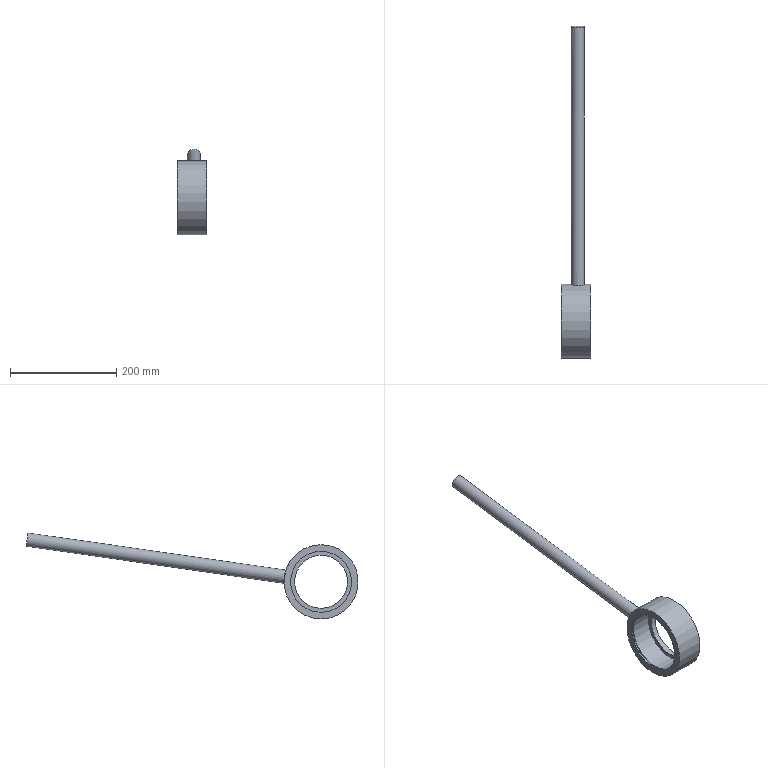Component | NX | DRIVE_ROD | 1 solid | 12 faces | box 55 x 626.09 x 161.96 mm | volume 538437 mm3 | cylinder 6 | plane 6 | commonest cylinder face diameters 115 x2 140 x1 100 x1 119 x1 25 x1
STEP:
#1=CARTESIAN_POINT('',(0.,0.,0.));
#2=DIRECTION('',(0.,0.,1.));
#3=DIRECTION('',(1.,0.,0.));
#4=AXIS2_PLACEMENT_3D('',#1,#2,#3);
#5=CARTESIAN_POINT('',(1368.754,222.349,548.477));
#6=VERTEX_POINT('',#5);
#7=CARTESIAN_POINT('',(1368.754,222.349,478.477));
#8=DIRECTION('',(1.,0.,0.));
#9=DIRECTION('',(0.,0.,1.));
#10=AXIS2_PLACEMENT_3D('',#7,#8,#9);
#11=CIRCLE('',#10,70.);
#12=CARTESIAN_POINT('',(1368.754,222.349,478.477));
#13=DIRECTION('',(-1.,0.,0.));
#14=DIRECTION('',(0.,0.,1.));
#15=AXIS2_PLACEMENT_3D('',#12,#13,#14);
#16=CYLINDRICAL_SURFACE('',#15,70.);
#17=CARTESIAN_POINT('',(6.283,0.));
#18=DIRECTION('',(-1.,0.));
#19=VECTOR('',#18,1.);
#20=LINE('',#17,#19);
#21=(GEOMETRIC_REPRESENTATION_CONTEXT(2)PARAMETRIC_REPRESENTATION_CONTEXT()REPRESENTATION_CONTEXT('',''));
#22=DEFINITIONAL_REPRESENTATION('',(#20),#21);
#23=PCURVE('',#16,#22);
#24=CARTESIAN_POINT('',(1368.754,222.349,478.477));
#25=DIRECTION('',(1.,0.,0.));
#26=DIRECTION('',(0.,0.,-1.));
#27=AXIS2_PLACEMENT_3D('',#24,#25,#26);
#28=PLANE('',#27);
#29=CARTESIAN_POINT('',(0.,0.));
#30=DIRECTION('',(-1.,0.));
#31=AXIS2_PLACEMENT_2D('',#29,#30);
#32=CIRCLE('',#31,70.);
#33=(GEOMETRIC_REPRESENTATION_CONTEXT(2)PARAMETRIC_REPRESENTATION_CONTEXT()REPRESENTATION_CONTEXT('',''));
#34=DEFINITIONAL_REPRESENTATION('',(#32),#33);
#35=PCURVE('',#28,#34);
#36=SURFACE_CURVE('',#11,(#23,#35),.PCURVE_S1.);
#37=EDGE_CURVE('',#6,#6,#36,.T.);
#38=ORIENTED_EDGE('',*,*,#37,.F.);
#39=CARTESIAN_POINT('',(1313.754,222.349,548.477));
#40=VERTEX_POINT('',#39);
#41=CARTESIAN_POINT('',(1368.754,222.349,548.477));
#42=CARTESIAN_POINT('',(1313.754,222.349,548.477));
#43=B_SPLINE_CURVE_WITH_KNOTS('',1,(#41,#42),.UNSPECIFIED.,.F.,.F.,(2,2),(0.,55.),.PIECEWISE_BEZIER_KNOTS.);
#44=CARTESIAN_POINT('',(6.283,0.));
#45=DIRECTION('',(0.,1.));
#46=VECTOR('',#45,1.);
#47=LINE('',#44,#46);
#48=(GEOMETRIC_REPRESENTATION_CONTEXT(2)PARAMETRIC_REPRESENTATION_CONTEXT()REPRESENTATION_CONTEXT('',''));
#49=DEFINITIONAL_REPRESENTATION('',(#47),#48);
#50=PCURVE('',#16,#49);
#51=CARTESIAN_POINT('',(0.,0.));
#52=DIRECTION('',(0.,1.));
#53=VECTOR('',#52,1.);
#54=LINE('',#51,#53);
#55=(GEOMETRIC_REPRESENTATION_CONTEXT(2)PARAMETRIC_REPRESENTATION_CONTEXT()REPRESENTATION_CONTEXT('',''));
#56=DEFINITIONAL_REPRESENTATION('',(#54),#55);
#57=PCURVE('',#16,#56);
#58=SEAM_CURVE('',#43,(#50,#57),.PCURVE_S1.);
#59=EDGE_CURVE('',#6,#40,#58,.T.);
#60=ORIENTED_EDGE('',*,*,#59,.T.);
#61=CARTESIAN_POINT('',(1313.754,222.349,478.477));
#62=DIRECTION('',(1.,0.,0.));
#63=DIRECTION('',(0.,0.,1.));
#64=AXIS2_PLACEMENT_3D('',#61,#62,#63);
#65=CIRCLE('',#64,70.);
#66=CARTESIAN_POINT('',(6.283,55.));
#67=DIRECTION('',(-1.,0.));
#68=VECTOR('',#67,1.);
#69=LINE('',#66,#68);
#70=(GEOMETRIC_REPRESENTATION_CONTEXT(2)PARAMETRIC_REPRESENTATION_CONTEXT()REPRESENTATION_CONTEXT('',''));
#71=DEFINITIONAL_REPRESENTATION('',(#69),#70);
#72=PCURVE('',#16,#71);
#73=CARTESIAN_POINT('',(1313.754,222.349,478.477));
#74=DIRECTION('',(1.,0.,0.));
#75=DIRECTION('',(0.,0.,-1.));
#76=AXIS2_PLACEMENT_3D('',#73,#74,#75);
#77=PLANE('',#76);
#78=CARTESIAN_POINT('',(0.,0.));
#79=DIRECTION('',(-1.,0.));
#80=AXIS2_PLACEMENT_2D('',#78,#79);
#81=CIRCLE('',#80,70.);
#82=(GEOMETRIC_REPRESENTATION_CONTEXT(2)PARAMETRIC_REPRESENTATION_CONTEXT()REPRESENTATION_CONTEXT('',''));
#83=DEFINITIONAL_REPRESENTATION('',(#81),#82);
#84=PCURVE('',#77,#83);
#85=SURFACE_CURVE('',#65,(#72,#84),.PCURVE_S1.);
#86=EDGE_CURVE('',#40,#40,#85,.T.);
#87=ORIENTED_EDGE('',*,*,#86,.T.);
#88=ORIENTED_EDGE('',*,*,#59,.F.);
#89=EDGE_LOOP('',(#38,#60,#87,#88));
#90=FACE_BOUND('',#89,.T.);
#91=CARTESIAN_POINT('',(1344.754,288.749,500.638));
#92=VERTEX_POINT('',#91);
#93=CARTESIAN_POINT('',(1341.444,288.749,500.638));
#94=CARTESIAN_POINT('',(1348.065,288.749,500.638));
#95=CARTESIAN_POINT('',(1351.293,289.212,499.33));
#96=CARTESIAN_POINT('',(1355.895,290.446,494.857));
#97=CARTESIAN_POINT('',(1357.252,291.173,491.667));
#98=CARTESIAN_POINT('',(1357.256,292.103,485.197));
#99=CARTESIAN_POINT('',(1355.921,292.303,481.944));
#100=CARTESIAN_POINT('',(1351.269,292.378,477.253));
#101=CARTESIAN_POINT('',(1348.026,292.302,475.893));
#102=CARTESIAN_POINT('',(1341.493,292.302,475.89));
#103=CARTESIAN_POINT('',(1338.23,292.378,477.267));
#104=CARTESIAN_POINT('',(1333.617,292.304,481.908));
#105=CARTESIAN_POINT('',(1332.257,292.109,485.146));
#106=CARTESIAN_POINT('',(1332.252,291.171,491.685));
#107=CARTESIAN_POINT('',(1333.611,290.447,494.851));
#108=CARTESIAN_POINT('',(1338.207,289.213,499.324));
#109=CARTESIAN_POINT('',(1341.444,288.749,500.638));
#110=CARTESIAN_POINT('',(1348.065,288.749,500.638));
#111=B_SPLINE_CURVE_WITH_KNOTS('',3,(#93,#94,#95,#96,#97,#98,#99,#100,#101,#102,#103,#104,#105,#106,#107,#108,#109,#110),.UNSPECIFIED.,.T.,.F.,(2,2,2,2,2,2,2,2,2,2,2),(-0.125,0.,0.125,0.25,0.375,0.5,0.625,0.75,0.875,1.,1.125),.UNSPECIFIED.);
#112=CARTESIAN_POINT('',(1.249,24.));
#113=CARTESIAN_POINT('',(1.249,23.398));
#114=CARTESIAN_POINT('',(1.25,22.2));
#115=CARTESIAN_POINT('',(1.256,20.449));
#116=CARTESIAN_POINT('',(1.265,18.775));
#117=CARTESIAN_POINT('',(1.277,17.21));
#118=CARTESIAN_POINT('',(1.292,15.782));
#119=CARTESIAN_POINT('',(1.311,14.524));
#120=CARTESIAN_POINT('',(1.331,13.462));
#121=CARTESIAN_POINT('',(1.354,12.609));
#122=CARTESIAN_POINT('',(1.378,11.98));
#123=CARTESIAN_POINT('',(1.403,11.591));
#124=CARTESIAN_POINT('',(1.428,11.455));
#125=CARTESIAN_POINT('',(1.454,11.587));
#126=CARTESIAN_POINT('',(1.478,11.972));
#127=CARTESIAN_POINT('',(1.502,12.596));
#128=CARTESIAN_POINT('',(1.525,13.448));
#129=CARTESIAN_POINT('',(1.546,14.515));
#130=CARTESIAN_POINT('',(1.564,15.788));
#131=CARTESIAN_POINT('',(1.579,17.226));
#132=CARTESIAN_POINT('',(1.592,18.799));
#133=CARTESIAN_POINT('',(1.601,20.472));
#134=CARTESIAN_POINT('',(1.606,22.215));
#135=CARTESIAN_POINT('',(1.608,23.995));
#136=CARTESIAN_POINT('',(1.606,25.777));
#137=CARTESIAN_POINT('',(1.601,27.523));
#138=CARTESIAN_POINT('',(1.592,29.199));
#139=CARTESIAN_POINT('',(1.579,30.772));
#140=CARTESIAN_POINT('',(1.564,32.208));
#141=CARTESIAN_POINT('',(1.546,33.469));
#142=CARTESIAN_POINT('',(1.525,34.533));
#143=CARTESIAN_POINT('',(1.503,35.388));
#144=CARTESIAN_POINT('',(1.479,36.018));
#145=CARTESIAN_POINT('',(1.454,36.409));
#146=CARTESIAN_POINT('',(1.428,36.545));
#147=CARTESIAN_POINT('',(1.403,36.411));
#148=CARTESIAN_POINT('',(1.378,36.023));
#149=CARTESIAN_POINT('',(1.354,35.395));
#150=CARTESIAN_POINT('',(1.331,34.542));
#151=CARTESIAN_POINT('',(1.311,33.481));
#152=CARTESIAN_POINT('',(1.293,32.225));
#153=CARTESIAN_POINT('',(1.277,30.796));
#154=CARTESIAN_POINT('',(1.265,29.229));
#155=CARTESIAN_POINT('',(1.256,27.553));
#156=CARTESIAN_POINT('',(1.25,25.801));
#157=CARTESIAN_POINT('',(1.249,24.602));
#158=CARTESIAN_POINT('',(1.249,24.));
#159=B_SPLINE_CURVE_WITH_KNOTS('',3,(#112,#113,#114,#115,#116,#117,#118,#119,#120,#121,#122,#123,#124,#125,#126,#127,#128,#129,#130,#131,#132,#133,#134,#135,#136,#137,#138,#139,#140,#141,#142,#143,#144,#145,#146,#147,#148,#149,#150,#151,#152,#153,#154,#155,#156,#157,#158),.UNSPECIFIED.,.T.,.F.,(4,1,1,1,1,1,1,1,1,1,1,1,1,1,1,1,1,1,1,1,1,1,1,1,1,1,1,1,1,1,1,1,1,1,1,1,1,1,1,1,1,1,1,1,4),(0.,0.02273,0.04545,0.06818,0.09091,0.1136,0.1364,0.1591,0.1818,0.2045,0.2273,0.25,0.2727,0.2955,0.3182,0.3409,0.3636,0.3864,0.4091,0.4318,0.4545,0.4773,0.5,0.5227,0.5455,0.5682,0.5909,0.6136,0.6364,0.6591,0.6818,0.7045,0.7273,0.75,0.7727,0.7955,0.8182,0.8409,0.8636,0.8864,0.9091,0.9318,0.9545,0.9773,1.),.QUASI_UNIFORM_KNOTS.);
#160=(GEOMETRIC_REPRESENTATION_CONTEXT(2)PARAMETRIC_REPRESENTATION_CONTEXT()REPRESENTATION_CONTEXT('',''));
#161=DEFINITIONAL_REPRESENTATION('',(#159),#160);
#162=PCURVE('',#16,#161);
#163=CARTESIAN_POINT('',(1344.754,776.666,558.06));
#164=DIRECTION('',(0.,0.9899,0.1421));
#165=DIRECTION('',(0.,-0.1421,0.9899));
#166=AXIS2_PLACEMENT_3D('',#163,#164,#165);
#167=CYLINDRICAL_SURFACE('',#166,12.5);
#168=CARTESIAN_POINT('',(0.,-491.125));
#169=CARTESIAN_POINT('',(0.04812,-491.125));
#170=CARTESIAN_POINT('',(0.144,-491.107));
#171=CARTESIAN_POINT('',(0.2872,-491.035));
#172=CARTESIAN_POINT('',(0.43,-490.928));
#173=CARTESIAN_POINT('',(0.5725,-490.793));
#174=CARTESIAN_POINT('',(0.7145,-490.641));
#175=CARTESIAN_POINT('',(0.8565,-490.479));
#176=CARTESIAN_POINT('',(0.9989,-490.328));
#177=CARTESIAN_POINT('',(1.142,-490.195));
#178=CARTESIAN_POINT('',(1.285,-490.089));
#179=CARTESIAN_POINT('',(1.428,-490.018));
#180=CARTESIAN_POINT('',(1.57,-489.991));
#181=CARTESIAN_POINT('',(1.713,-490.017));
#182=CARTESIAN_POINT('',(1.855,-490.087));
#183=CARTESIAN_POINT('',(1.998,-490.193));
#184=CARTESIAN_POINT('',(2.141,-490.326));
#185=CARTESIAN_POINT('',(2.284,-490.478));
#186=CARTESIAN_POINT('',(2.428,-490.642));
#187=CARTESIAN_POINT('',(2.571,-490.794));
#188=CARTESIAN_POINT('',(2.714,-490.929));
#189=CARTESIAN_POINT('',(2.856,-491.036));
#190=CARTESIAN_POINT('',(2.999,-491.107));
#191=CARTESIAN_POINT('',(3.141,-491.134));
#192=CARTESIAN_POINT('',(3.284,-491.107));
#193=CARTESIAN_POINT('',(3.427,-491.036));
#194=CARTESIAN_POINT('',(3.57,-490.928));
#195=CARTESIAN_POINT('',(3.713,-490.794));
#196=CARTESIAN_POINT('',(3.855,-490.642));
#197=CARTESIAN_POINT('',(3.997,-490.48));
#198=CARTESIAN_POINT('',(4.139,-490.329));
#199=CARTESIAN_POINT('',(4.282,-490.195));
#200=CARTESIAN_POINT('',(4.425,-490.089));
#201=CARTESIAN_POINT('',(4.568,-490.018));
#202=CARTESIAN_POINT('',(4.712,-489.991));
#203=CARTESIAN_POINT('',(4.855,-490.017));
#204=CARTESIAN_POINT('',(4.999,-490.088));
#205=CARTESIAN_POINT('',(5.141,-490.194));
#206=CARTESIAN_POINT('',(5.284,-490.328));
#207=CARTESIAN_POINT('',(5.426,-490.479));
#208=CARTESIAN_POINT('',(5.568,-490.64));
#209=CARTESIAN_POINT('',(5.71,-490.792));
#210=CARTESIAN_POINT('',(5.853,-490.927));
#211=CARTESIAN_POINT('',(5.996,-491.035));
#212=CARTESIAN_POINT('',(6.139,-491.107));
#213=CARTESIAN_POINT('',(6.235,-491.125));
#214=CARTESIAN_POINT('',(6.283,-491.125));
#215=B_SPLINE_CURVE_WITH_KNOTS('',3,(#168,#169,#170,#171,#172,#173,#174,#175,#176,#177,#178,#179,#180,#181,#182,#183,#184,#185,#186,#187,#188,#189,#190,#191,#192,#193,#194,#195,#196,#197,#198,#199,#200,#201,#202,#203,#204,#205,#206,#207,#208,#209,#210,#211,#212,#213,#214),.UNSPECIFIED.,.F.,.F.,(4,1,1,1,1,1,1,1,1,1,1,1,1,1,1,1,1,1,1,1,1,1,1,1,1,1,1,1,1,1,1,1,1,1,1,1,1,1,1,1,1,1,1,1,4),(0.,0.02273,0.04545,0.06818,0.09091,0.1136,0.1364,0.1591,0.1818,0.2045,0.2273,0.25,0.2727,0.2955,0.3182,0.3409,0.3636,0.3864,0.4091,0.4318,0.4545,0.4773,0.5,0.5227,0.5455,0.5682,0.5909,0.6136,0.6364,0.6591,0.6818,0.7045,0.7273,0.75,0.7727,0.7955,0.8182,0.8409,0.8636,0.8864,0.9091,0.9318,0.9545,0.9773,1.),.QUASI_UNIFORM_KNOTS.);
#216=(GEOMETRIC_REPRESENTATION_CONTEXT(2)PARAMETRIC_REPRESENTATION_CONTEXT()REPRESENTATION_CONTEXT('',''));
#217=DEFINITIONAL_REPRESENTATION('',(#215),#216);
#218=PCURVE('',#167,#217);
#219=SURFACE_CURVE('',#111,(#162,#218),.PCURVE_S1.);
#220=EDGE_CURVE('',#92,#92,#219,.T.);
#221=ORIENTED_EDGE('',*,*,#220,.F.);
#222=EDGE_LOOP('',(#221));
#223=FACE_BOUND('',#222,.T.);
#224=ADVANCED_FACE('',(#90,#223),#16,.T.);
#225=CARTESIAN_POINT('',(1358.754,222.349,420.977));
#226=VERTEX_POINT('',#225);
#227=CARTESIAN_POINT('',(1358.754,222.349,478.477));
#228=DIRECTION('',(1.,0.,0.));
#229=DIRECTION('',(0.,0.,-1.));
#230=AXIS2_PLACEMENT_3D('',#227,#228,#229);
#231=CIRCLE('',#230,57.5);
#232=CARTESIAN_POINT('',(1313.754,222.349,478.477));
#233=DIRECTION('',(1.,0.,0.));
#234=DIRECTION('',(0.,0.,-1.));
#235=AXIS2_PLACEMENT_3D('',#232,#233,#234);
#236=CYLINDRICAL_SURFACE('',#235,57.5);
#237=CARTESIAN_POINT('',(0.,45.));
#238=DIRECTION('',(1.,0.));
#239=VECTOR('',#238,1.);
#240=LINE('',#237,#239);
#241=(GEOMETRIC_REPRESENTATION_CONTEXT(2)PARAMETRIC_REPRESENTATION_CONTEXT()REPRESENTATION_CONTEXT('',''));
#242=DEFINITIONAL_REPRESENTATION('',(#240),#241);
#243=PCURVE('',#236,#242);
#244=CARTESIAN_POINT('',(1358.754,222.349,478.477));
#245=DIRECTION('',(1.,0.,0.));
#246=DIRECTION('',(0.,0.,-1.));
#247=AXIS2_PLACEMENT_3D('',#244,#245,#246);
#248=PLANE('',#247);
#249=CARTESIAN_POINT('',(0.,0.));
#250=DIRECTION('',(1.,0.));
#251=AXIS2_PLACEMENT_2D('',#249,#250);
#252=CIRCLE('',#251,57.5);
#253=(GEOMETRIC_REPRESENTATION_CONTEXT(2)PARAMETRIC_REPRESENTATION_CONTEXT()REPRESENTATION_CONTEXT('',''));
#254=DEFINITIONAL_REPRESENTATION('',(#252),#253);
#255=PCURVE('',#248,#254);
#256=SURFACE_CURVE('',#231,(#243,#255),.PCURVE_S1.);
#257=EDGE_CURVE('',#226,#226,#256,.T.);
#258=ORIENTED_EDGE('',*,*,#257,.F.);
#259=CARTESIAN_POINT('',(1318.754,222.349,420.977));
#260=VERTEX_POINT('',#259);
#261=CARTESIAN_POINT('',(1318.754,222.349,420.977));
#262=CARTESIAN_POINT('',(1358.754,222.349,420.977));
#263=B_SPLINE_CURVE_WITH_KNOTS('',1,(#261,#262),.UNSPECIFIED.,.F.,.F.,(2,2),(5.,45.),.PIECEWISE_BEZIER_KNOTS.);
#264=CARTESIAN_POINT('',(0.,0.));
#265=DIRECTION('',(0.,1.));
#266=VECTOR('',#265,1.);
#267=LINE('',#264,#266);
#268=(GEOMETRIC_REPRESENTATION_CONTEXT(2)PARAMETRIC_REPRESENTATION_CONTEXT()REPRESENTATION_CONTEXT('',''));
#269=DEFINITIONAL_REPRESENTATION('',(#267),#268);
#270=PCURVE('',#236,#269);
#271=CARTESIAN_POINT('',(6.283,0.));
#272=DIRECTION('',(0.,1.));
#273=VECTOR('',#272,1.);
#274=LINE('',#271,#273);
#275=(GEOMETRIC_REPRESENTATION_CONTEXT(2)PARAMETRIC_REPRESENTATION_CONTEXT()REPRESENTATION_CONTEXT('',''));
#276=DEFINITIONAL_REPRESENTATION('',(#274),#275);
#277=PCURVE('',#236,#276);
#278=SEAM_CURVE('',#263,(#270,#277),.PCURVE_S1.);
#279=EDGE_CURVE('',#260,#226,#278,.T.);
#280=ORIENTED_EDGE('',*,*,#279,.F.);
#281=CARTESIAN_POINT('',(1318.754,222.349,535.977));
#282=VERTEX_POINT('',#281);
#283=CARTESIAN_POINT('',(1318.754,222.349,478.477));
#284=DIRECTION('',(1.,0.,0.));
#285=DIRECTION('',(0.,0.,1.));
#286=AXIS2_PLACEMENT_3D('',#283,#284,#285);
#287=CIRCLE('',#286,57.5);
#288=CARTESIAN_POINT('',(-3.142,5.));
#289=DIRECTION('',(1.,0.));
#290=VECTOR('',#289,1.);
#291=LINE('',#288,#290);
#292=(GEOMETRIC_REPRESENTATION_CONTEXT(2)PARAMETRIC_REPRESENTATION_CONTEXT()REPRESENTATION_CONTEXT('',''));
#293=DEFINITIONAL_REPRESENTATION('',(#291),#292);
#294=PCURVE('',#236,#293);
#295=CARTESIAN_POINT('',(1318.754,222.349,478.477));
#296=DIRECTION('',(-1.,0.,0.));
#297=DIRECTION('',(0.,0.,1.));
#298=AXIS2_PLACEMENT_3D('',#295,#296,#297);
#299=PLANE('',#298);
#300=CARTESIAN_POINT('',(57.5,0.));
#301=CARTESIAN_POINT('',(57.5,-99.593));
#302=CARTESIAN_POINT('',(-28.75,-49.796));
#303=CARTESIAN_POINT('',(-115.,-0.));
#304=CARTESIAN_POINT('',(-28.75,49.796));
#305=CARTESIAN_POINT('',(57.5,99.593));
#306=CARTESIAN_POINT('',(57.5,0.));
#307=(BOUNDED_CURVE()B_SPLINE_CURVE(2,(#300,#301,#302,#303,#304,#305,#306),.UNSPECIFIED.,.T.,.F.)B_SPLINE_CURVE_WITH_KNOTS((1,2,2,2,2,1),(-2.094,0.,2.094,4.189,6.283,8.378),.UNSPECIFIED.)CURVE()GEOMETRIC_REPRESENTATION_ITEM()RATIONAL_B_SPLINE_CURVE((1.,0.5,1.,0.5,1.,0.5,1.))REPRESENTATION_ITEM(''));
#308=(GEOMETRIC_REPRESENTATION_CONTEXT(2)PARAMETRIC_REPRESENTATION_CONTEXT()REPRESENTATION_CONTEXT('',''));
#309=DEFINITIONAL_REPRESENTATION('',(#307),#308);
#310=PCURVE('',#299,#309);
#311=SURFACE_CURVE('',#287,(#294,#310),.PCURVE_S1.);
#312=EDGE_CURVE('',#260,#282,#311,.T.);
#313=ORIENTED_EDGE('',*,*,#312,.T.);
#314=CARTESIAN_POINT('',(1318.754,222.349,478.477));
#315=DIRECTION('',(1.,0.,0.));
#316=DIRECTION('',(0.,0.,1.));
#317=AXIS2_PLACEMENT_3D('',#314,#315,#316);
#318=CIRCLE('',#317,57.5);
#319=CARTESIAN_POINT('',(3.142,5.));
#320=DIRECTION('',(1.,0.));
#321=VECTOR('',#320,1.);
#322=LINE('',#319,#321);
#323=(GEOMETRIC_REPRESENTATION_CONTEXT(2)PARAMETRIC_REPRESENTATION_CONTEXT()REPRESENTATION_CONTEXT('',''));
#324=DEFINITIONAL_REPRESENTATION('',(#322),#323);
#325=PCURVE('',#236,#324);
#326=CARTESIAN_POINT('',(57.5,0.));
#327=CARTESIAN_POINT('',(57.5,-99.593));
#328=CARTESIAN_POINT('',(-28.75,-49.796));
#329=CARTESIAN_POINT('',(-115.,-0.));
#330=CARTESIAN_POINT('',(-28.75,49.796));
#331=CARTESIAN_POINT('',(57.5,99.593));
#332=CARTESIAN_POINT('',(57.5,0.));
#333=(BOUNDED_CURVE()B_SPLINE_CURVE(2,(#326,#327,#328,#329,#330,#331,#332),.UNSPECIFIED.,.T.,.F.)B_SPLINE_CURVE_WITH_KNOTS((1,2,2,2,2,1),(-2.094,0.,2.094,4.189,6.283,8.378),.UNSPECIFIED.)CURVE()GEOMETRIC_REPRESENTATION_ITEM()RATIONAL_B_SPLINE_CURVE((1.,0.5,1.,0.5,1.,0.5,1.))REPRESENTATION_ITEM(''));
#334=(GEOMETRIC_REPRESENTATION_CONTEXT(2)PARAMETRIC_REPRESENTATION_CONTEXT()REPRESENTATION_CONTEXT('',''));
#335=DEFINITIONAL_REPRESENTATION('',(#333),#334);
#336=PCURVE('',#299,#335);
#337=SURFACE_CURVE('',#318,(#325,#336),.PCURVE_S1.);
#338=EDGE_CURVE('',#282,#260,#337,.T.);
#339=ORIENTED_EDGE('',*,*,#338,.T.);
#340=ORIENTED_EDGE('',*,*,#279,.T.);
#341=EDGE_LOOP('',(#258,#280,#313,#339,#340));
#342=FACE_BOUND('',#341,.F.);
#343=ADVANCED_FACE('',(#342),#236,.F.);
#344=CARTESIAN_POINT('',(1358.754,222.349,428.477));
#345=VERTEX_POINT('',#344);
#346=CARTESIAN_POINT('',(1358.754,222.349,528.477));
#347=VERTEX_POINT('',#346);
#348=CARTESIAN_POINT('',(1358.754,222.349,478.477));
#349=DIRECTION('',(1.,0.,0.));
#350=DIRECTION('',(0.,0.,-1.));
#351=AXIS2_PLACEMENT_3D('',#348,#349,#350);
#352=CIRCLE('',#351,50.);
#353=CARTESIAN_POINT('',(1368.754,222.349,478.477));
#354=DIRECTION('',(-1.,0.,0.));
#355=DIRECTION('',(0.,0.,1.));
#356=AXIS2_PLACEMENT_3D('',#353,#354,#355);
#357=CYLINDRICAL_SURFACE('',#356,50.);
#358=CARTESIAN_POINT('',(3.142,10.));
#359=DIRECTION('',(-1.,0.));
#360=VECTOR('',#359,1.);
#361=LINE('',#358,#360);
#362=(GEOMETRIC_REPRESENTATION_CONTEXT(2)PARAMETRIC_REPRESENTATION_CONTEXT()REPRESENTATION_CONTEXT('',''));
#363=DEFINITIONAL_REPRESENTATION('',(#361),#362);
#364=PCURVE('',#357,#363);
#365=CARTESIAN_POINT('',(0.,0.));
#366=DIRECTION('',(1.,0.));
#367=AXIS2_PLACEMENT_2D('',#365,#366);
#368=CIRCLE('',#367,50.);
#369=(GEOMETRIC_REPRESENTATION_CONTEXT(2)PARAMETRIC_REPRESENTATION_CONTEXT()REPRESENTATION_CONTEXT('',''));
#370=DEFINITIONAL_REPRESENTATION('',(#368),#369);
#371=PCURVE('',#248,#370);
#372=SURFACE_CURVE('',#352,(#364,#371),.PCURVE_S1.);
#373=EDGE_CURVE('',#345,#347,#372,.T.);
#374=ORIENTED_EDGE('',*,*,#373,.T.);
#375=CARTESIAN_POINT('',(1368.754,222.349,528.477));
#376=VERTEX_POINT('',#375);
#377=CARTESIAN_POINT('',(1368.754,222.349,528.477));
#378=CARTESIAN_POINT('',(1358.754,222.349,528.477));
#379=B_SPLINE_CURVE_WITH_KNOTS('',1,(#377,#378),.UNSPECIFIED.,.F.,.F.,(2,2),(0.,10.),.PIECEWISE_BEZIER_KNOTS.);
#380=CARTESIAN_POINT('',(0.,0.));
#381=DIRECTION('',(0.,1.));
#382=VECTOR('',#381,1.);
#383=LINE('',#380,#382);
#384=(GEOMETRIC_REPRESENTATION_CONTEXT(2)PARAMETRIC_REPRESENTATION_CONTEXT()REPRESENTATION_CONTEXT('',''));
#385=DEFINITIONAL_REPRESENTATION('',(#383),#384);
#386=PCURVE('',#357,#385);
#387=CARTESIAN_POINT('',(6.283,0.));
#388=DIRECTION('',(0.,1.));
#389=VECTOR('',#388,1.);
#390=LINE('',#387,#389);
#391=(GEOMETRIC_REPRESENTATION_CONTEXT(2)PARAMETRIC_REPRESENTATION_CONTEXT()REPRESENTATION_CONTEXT('',''));
#392=DEFINITIONAL_REPRESENTATION('',(#390),#391);
#393=PCURVE('',#357,#392);
#394=SEAM_CURVE('',#379,(#386,#393),.PCURVE_S1.);
#395=EDGE_CURVE('',#376,#347,#394,.T.);
#396=ORIENTED_EDGE('',*,*,#395,.F.);
#397=CARTESIAN_POINT('',(1368.754,222.349,478.477));
#398=DIRECTION('',(1.,0.,0.));
#399=DIRECTION('',(0.,0.,1.));
#400=AXIS2_PLACEMENT_3D('',#397,#398,#399);
#401=CIRCLE('',#400,50.);
#402=CARTESIAN_POINT('',(6.283,0.));
#403=DIRECTION('',(-1.,0.));
#404=VECTOR('',#403,1.);
#405=LINE('',#402,#404);
#406=(GEOMETRIC_REPRESENTATION_CONTEXT(2)PARAMETRIC_REPRESENTATION_CONTEXT()REPRESENTATION_CONTEXT('',''));
#407=DEFINITIONAL_REPRESENTATION('',(#405),#406);
#408=PCURVE('',#357,#407);
#409=CARTESIAN_POINT('',(0.,0.));
#410=DIRECTION('',(-1.,0.));
#411=AXIS2_PLACEMENT_2D('',#409,#410);
#412=CIRCLE('',#411,50.);
#413=(GEOMETRIC_REPRESENTATION_CONTEXT(2)PARAMETRIC_REPRESENTATION_CONTEXT()REPRESENTATION_CONTEXT('',''));
#414=DEFINITIONAL_REPRESENTATION('',(#412),#413);
#415=PCURVE('',#28,#414);
#416=SURFACE_CURVE('',#401,(#408,#415),.PCURVE_S1.);
#417=EDGE_CURVE('',#376,#376,#416,.T.);
#418=ORIENTED_EDGE('',*,*,#417,.F.);
#419=ORIENTED_EDGE('',*,*,#395,.T.);
#420=CARTESIAN_POINT('',(1358.754,222.349,478.477));
#421=DIRECTION('',(1.,0.,0.));
#422=DIRECTION('',(0.,0.,-1.));
#423=AXIS2_PLACEMENT_3D('',#420,#421,#422);
#424=CIRCLE('',#423,50.);
#425=CARTESIAN_POINT('',(9.425,10.));
#426=DIRECTION('',(-1.,0.));
#427=VECTOR('',#426,1.);
#428=LINE('',#425,#427);
#429=(GEOMETRIC_REPRESENTATION_CONTEXT(2)PARAMETRIC_REPRESENTATION_CONTEXT()REPRESENTATION_CONTEXT('',''));
#430=DEFINITIONAL_REPRESENTATION('',(#428),#429);
#431=PCURVE('',#357,#430);
#432=CARTESIAN_POINT('',(0.,0.));
#433=DIRECTION('',(1.,0.));
#434=AXIS2_PLACEMENT_2D('',#432,#433);
#435=CIRCLE('',#434,50.);
#436=(GEOMETRIC_REPRESENTATION_CONTEXT(2)PARAMETRIC_REPRESENTATION_CONTEXT()REPRESENTATION_CONTEXT('',''));
#437=DEFINITIONAL_REPRESENTATION('',(#435),#436);
#438=PCURVE('',#248,#437);
#439=SURFACE_CURVE('',#424,(#431,#438),.PCURVE_S1.);
#440=EDGE_CURVE('',#347,#345,#439,.T.);
#441=ORIENTED_EDGE('',*,*,#440,.T.);
#442=EDGE_LOOP('',(#374,#396,#418,#419,#441));
#443=FACE_BOUND('',#442,.F.);
#444=ADVANCED_FACE('',(#443),#357,.F.);
#445=ORIENTED_EDGE('',*,*,#37,.T.);
#446=EDGE_LOOP('',(#445));
#447=FACE_BOUND('',#446,.T.);
#448=ORIENTED_EDGE('',*,*,#417,.F.);
#449=EDGE_LOOP('',(#448));
#450=FACE_BOUND('',#449,.T.);
#451=ADVANCED_FACE('',(#447,#450),#28,.T.);
#452=CARTESIAN_POINT('',(1313.754,222.349,420.977));
#453=VERTEX_POINT('',#452);
#454=CARTESIAN_POINT('',(1313.754,222.349,478.477));
#455=DIRECTION('',(1.,0.,0.));
#456=DIRECTION('',(0.,0.,-1.));
#457=AXIS2_PLACEMENT_3D('',#454,#455,#456);
#458=CIRCLE('',#457,57.5);
#459=CARTESIAN_POINT('',(0.,0.));
#460=DIRECTION('',(1.,0.));
#461=AXIS2_PLACEMENT_2D('',#459,#460);
#462=CIRCLE('',#461,57.5);
#463=(GEOMETRIC_REPRESENTATION_CONTEXT(2)PARAMETRIC_REPRESENTATION_CONTEXT()REPRESENTATION_CONTEXT('',''));
#464=DEFINITIONAL_REPRESENTATION('',(#462),#463);
#465=PCURVE('',#77,#464);
#466=CARTESIAN_POINT('',(1313.754,222.349,478.477));
#467=DIRECTION('',(1.,0.,0.));
#468=DIRECTION('',(0.,0.,-1.));
#469=AXIS2_PLACEMENT_3D('',#466,#467,#468);
#470=CYLINDRICAL_SURFACE('',#469,57.5);
#471=CARTESIAN_POINT('',(0.,0.));
#472=DIRECTION('',(1.,0.));
#473=VECTOR('',#472,1.);
#474=LINE('',#471,#473);
#475=(GEOMETRIC_REPRESENTATION_CONTEXT(2)PARAMETRIC_REPRESENTATION_CONTEXT()REPRESENTATION_CONTEXT('',''));
#476=DEFINITIONAL_REPRESENTATION('',(#474),#475);
#477=PCURVE('',#470,#476);
#478=SURFACE_CURVE('',#458,(#465,#477),.PCURVE_S1.);
#479=EDGE_CURVE('',#453,#453,#478,.T.);
#480=ORIENTED_EDGE('',*,*,#479,.T.);
#481=EDGE_LOOP('',(#480));
#482=FACE_BOUND('',#481,.T.);
#483=ORIENTED_EDGE('',*,*,#86,.F.);
#484=EDGE_LOOP('',(#483));
#485=FACE_BOUND('',#484,.T.);
#486=ADVANCED_FACE('',(#482,#485),#77,.F.);
#487=ORIENTED_EDGE('',*,*,#373,.T.);
#488=ORIENTED_EDGE('',*,*,#440,.T.);
#489=EDGE_LOOP('',(#487,#488));
#490=FACE_BOUND('',#489,.T.);
#491=ORIENTED_EDGE('',*,*,#257,.F.);
#492=EDGE_LOOP('',(#491));
#493=FACE_BOUND('',#492,.T.);
#494=ADVANCED_FACE('',(#490,#493),#248,.F.);
#495=CARTESIAN_POINT('',(1314.754,222.349,420.977));
#496=VERTEX_POINT('',#495);
#497=CARTESIAN_POINT('',(1314.754,222.349,535.977));
#498=VERTEX_POINT('',#497);
#499=CARTESIAN_POINT('',(1314.754,222.349,478.477));
#500=DIRECTION('',(1.,0.,0.));
#501=DIRECTION('',(0.,0.,1.));
#502=AXIS2_PLACEMENT_3D('',#499,#500,#501);
#503=CIRCLE('',#502,57.5);
#504=CARTESIAN_POINT('',(-3.142,1.));
#505=DIRECTION('',(1.,0.));
#506=VECTOR('',#505,1.);
#507=LINE('',#504,#506);
#508=(GEOMETRIC_REPRESENTATION_CONTEXT(2)PARAMETRIC_REPRESENTATION_CONTEXT()REPRESENTATION_CONTEXT('',''));
#509=DEFINITIONAL_REPRESENTATION('',(#507),#508);
#510=PCURVE('',#470,#509);
#511=CARTESIAN_POINT('',(1314.754,222.349,478.477));
#512=DIRECTION('',(-1.,0.,0.));
#513=DIRECTION('',(0.,0.,1.));
#514=AXIS2_PLACEMENT_3D('',#511,#512,#513);
#515=PLANE('',#514);
#516=CARTESIAN_POINT('',(57.5,0.));
#517=CARTESIAN_POINT('',(57.5,-99.593));
#518=CARTESIAN_POINT('',(-28.75,-49.796));
#519=CARTESIAN_POINT('',(-115.,-0.));
#520=CARTESIAN_POINT('',(-28.75,49.796));
#521=CARTESIAN_POINT('',(57.5,99.593));
#522=CARTESIAN_POINT('',(57.5,0.));
#523=(BOUNDED_CURVE()B_SPLINE_CURVE(2,(#516,#517,#518,#519,#520,#521,#522),.UNSPECIFIED.,.T.,.F.)B_SPLINE_CURVE_WITH_KNOTS((1,2,2,2,2,1),(-2.094,0.,2.094,4.189,6.283,8.378),.UNSPECIFIED.)CURVE()GEOMETRIC_REPRESENTATION_ITEM()RATIONAL_B_SPLINE_CURVE((1.,0.5,1.,0.5,1.,0.5,1.))REPRESENTATION_ITEM(''));
#524=(GEOMETRIC_REPRESENTATION_CONTEXT(2)PARAMETRIC_REPRESENTATION_CONTEXT()REPRESENTATION_CONTEXT('',''));
#525=DEFINITIONAL_REPRESENTATION('',(#523),#524);
#526=PCURVE('',#515,#525);
#527=SURFACE_CURVE('',#503,(#510,#526),.PCURVE_S1.);
#528=EDGE_CURVE('',#496,#498,#527,.T.);
#529=ORIENTED_EDGE('',*,*,#528,.F.);
#530=CARTESIAN_POINT('',(1313.754,222.349,420.977));
#531=CARTESIAN_POINT('',(1314.754,222.349,420.977));
#532=B_SPLINE_CURVE_WITH_KNOTS('',1,(#530,#531),.UNSPECIFIED.,.F.,.F.,(2,2),(0.,1.),.PIECEWISE_BEZIER_KNOTS.);
#533=CARTESIAN_POINT('',(0.,0.));
#534=DIRECTION('',(0.,1.));
#535=VECTOR('',#534,1.);
#536=LINE('',#533,#535);
#537=(GEOMETRIC_REPRESENTATION_CONTEXT(2)PARAMETRIC_REPRESENTATION_CONTEXT()REPRESENTATION_CONTEXT('',''));
#538=DEFINITIONAL_REPRESENTATION('',(#536),#537);
#539=PCURVE('',#470,#538);
#540=CARTESIAN_POINT('',(6.283,0.));
#541=DIRECTION('',(0.,1.));
#542=VECTOR('',#541,1.);
#543=LINE('',#540,#542);
#544=(GEOMETRIC_REPRESENTATION_CONTEXT(2)PARAMETRIC_REPRESENTATION_CONTEXT()REPRESENTATION_CONTEXT('',''));
#545=DEFINITIONAL_REPRESENTATION('',(#543),#544);
#546=PCURVE('',#470,#545);
#547=SEAM_CURVE('',#532,(#539,#546),.PCURVE_S1.);
#548=EDGE_CURVE('',#453,#496,#547,.T.);
#549=ORIENTED_EDGE('',*,*,#548,.F.);
#550=ORIENTED_EDGE('',*,*,#479,.T.);
#551=ORIENTED_EDGE('',*,*,#548,.T.);
#552=CARTESIAN_POINT('',(1314.754,222.349,478.477));
#553=DIRECTION('',(1.,0.,0.));
#554=DIRECTION('',(0.,0.,1.));
#555=AXIS2_PLACEMENT_3D('',#552,#553,#554);
#556=CIRCLE('',#555,57.5);
#557=CARTESIAN_POINT('',(3.142,1.));
#558=DIRECTION('',(1.,0.));
#559=VECTOR('',#558,1.);
#560=LINE('',#557,#559);
#561=(GEOMETRIC_REPRESENTATION_CONTEXT(2)PARAMETRIC_REPRESENTATION_CONTEXT()REPRESENTATION_CONTEXT('',''));
#562=DEFINITIONAL_REPRESENTATION('',(#560),#561);
#563=PCURVE('',#470,#562);
#564=CARTESIAN_POINT('',(57.5,0.));
#565=CARTESIAN_POINT('',(57.5,-99.593));
#566=CARTESIAN_POINT('',(-28.75,-49.796));
#567=CARTESIAN_POINT('',(-115.,-0.));
#568=CARTESIAN_POINT('',(-28.75,49.796));
#569=CARTESIAN_POINT('',(57.5,99.593));
#570=CARTESIAN_POINT('',(57.5,0.));
#571=(BOUNDED_CURVE()B_SPLINE_CURVE(2,(#564,#565,#566,#567,#568,#569,#570),.UNSPECIFIED.,.T.,.F.)B_SPLINE_CURVE_WITH_KNOTS((1,2,2,2,2,1),(-2.094,0.,2.094,4.189,6.283,8.378),.UNSPECIFIED.)CURVE()GEOMETRIC_REPRESENTATION_ITEM()RATIONAL_B_SPLINE_CURVE((1.,0.5,1.,0.5,1.,0.5,1.))REPRESENTATION_ITEM(''));
#572=(GEOMETRIC_REPRESENTATION_CONTEXT(2)PARAMETRIC_REPRESENTATION_CONTEXT()REPRESENTATION_CONTEXT('',''));
#573=DEFINITIONAL_REPRESENTATION('',(#571),#572);
#574=PCURVE('',#515,#573);
#575=SURFACE_CURVE('',#556,(#563,#574),.PCURVE_S1.);
#576=EDGE_CURVE('',#498,#496,#575,.T.);
#577=ORIENTED_EDGE('',*,*,#576,.F.);
#578=EDGE_LOOP('',(#529,#549,#550,#551,#577));
#579=FACE_BOUND('',#578,.F.);
#580=ADVANCED_FACE('',(#579),#470,.F.);
#581=CARTESIAN_POINT('',(1318.754,281.849,478.477));
#582=VERTEX_POINT('',#581);
#583=CARTESIAN_POINT('',(1318.754,222.349,478.477));
#584=DIRECTION('',(1.,0.,0.));
#585=DIRECTION('',(0.,1.,0.));
#586=AXIS2_PLACEMENT_3D('',#583,#584,#585);
#587=CIRCLE('',#586,59.5);
#588=CARTESIAN_POINT('',(0.,59.5));
#589=CARTESIAN_POINT('',(103.057,59.5));
#590=CARTESIAN_POINT('',(51.529,-29.75));
#591=CARTESIAN_POINT('',(0.,-119.));
#592=CARTESIAN_POINT('',(-51.529,-29.75));
#593=CARTESIAN_POINT('',(-103.057,59.5));
#594=CARTESIAN_POINT('',(0.,59.5));
#595=(BOUNDED_CURVE()B_SPLINE_CURVE(2,(#588,#589,#590,#591,#592,#593,#594),.UNSPECIFIED.,.T.,.F.)B_SPLINE_CURVE_WITH_KNOTS((1,2,2,2,2,1),(-2.094,0.,2.094,4.189,6.283,8.378),.UNSPECIFIED.)CURVE()GEOMETRIC_REPRESENTATION_ITEM()RATIONAL_B_SPLINE_CURVE((1.,0.5,1.,0.5,1.,0.5,1.))REPRESENTATION_ITEM(''));
#596=(GEOMETRIC_REPRESENTATION_CONTEXT(2)PARAMETRIC_REPRESENTATION_CONTEXT()REPRESENTATION_CONTEXT('',''));
#597=DEFINITIONAL_REPRESENTATION('',(#595),#596);
#598=PCURVE('',#299,#597);
#599=CARTESIAN_POINT('',(1318.754,222.349,478.477));
#600=DIRECTION('',(-1.,0.,0.));
#601=DIRECTION('',(0.,0.,1.));
#602=AXIS2_PLACEMENT_3D('',#599,#600,#601);
#603=CYLINDRICAL_SURFACE('',#602,59.5);
#604=CARTESIAN_POINT('',(7.854,0.));
#605=DIRECTION('',(-1.,0.));
#606=VECTOR('',#605,1.);
#607=LINE('',#604,#606);
#608=(GEOMETRIC_REPRESENTATION_CONTEXT(2)PARAMETRIC_REPRESENTATION_CONTEXT()REPRESENTATION_CONTEXT('',''));
#609=DEFINITIONAL_REPRESENTATION('',(#607),#608);
#610=PCURVE('',#603,#609);
#611=SURFACE_CURVE('',#587,(#598,#610),.PCURVE_S1.);
#612=EDGE_CURVE('',#582,#582,#611,.T.);
#613=ORIENTED_EDGE('',*,*,#612,.F.);
#614=EDGE_LOOP('',(#613));
#615=FACE_BOUND('',#614,.T.);
#616=ORIENTED_EDGE('',*,*,#338,.T.);
#617=ORIENTED_EDGE('',*,*,#312,.T.);
#618=EDGE_LOOP('',(#616,#617));
#619=FACE_BOUND('',#618,.T.);
#620=ADVANCED_FACE('',(#615,#619),#299,.T.);
#621=CARTESIAN_POINT('',(1314.754,281.849,478.477));
#622=VERTEX_POINT('',#621);
#623=CARTESIAN_POINT('',(1314.754,222.349,478.477));
#624=DIRECTION('',(1.,0.,0.));
#625=DIRECTION('',(0.,1.,0.));
#626=AXIS2_PLACEMENT_3D('',#623,#624,#625);
#627=CIRCLE('',#626,59.5);
#628=CARTESIAN_POINT('',(0.,59.5));
#629=CARTESIAN_POINT('',(103.057,59.5));
#630=CARTESIAN_POINT('',(51.529,-29.75));
#631=CARTESIAN_POINT('',(0.,-119.));
#632=CARTESIAN_POINT('',(-51.529,-29.75));
#633=CARTESIAN_POINT('',(-103.057,59.5));
#634=CARTESIAN_POINT('',(0.,59.5));
#635=(BOUNDED_CURVE()B_SPLINE_CURVE(2,(#628,#629,#630,#631,#632,#633,#634),.UNSPECIFIED.,.T.,.F.)B_SPLINE_CURVE_WITH_KNOTS((1,2,2,2,2,1),(-2.094,0.,2.094,4.189,6.283,8.378),.UNSPECIFIED.)CURVE()GEOMETRIC_REPRESENTATION_ITEM()RATIONAL_B_SPLINE_CURVE((1.,0.5,1.,0.5,1.,0.5,1.))REPRESENTATION_ITEM(''));
#636=(GEOMETRIC_REPRESENTATION_CONTEXT(2)PARAMETRIC_REPRESENTATION_CONTEXT()REPRESENTATION_CONTEXT('',''));
#637=DEFINITIONAL_REPRESENTATION('',(#635),#636);
#638=PCURVE('',#515,#637);
#639=CARTESIAN_POINT('',(7.854,4.));
#640=DIRECTION('',(-1.,0.));
#641=VECTOR('',#640,1.);
#642=LINE('',#639,#641);
#643=(GEOMETRIC_REPRESENTATION_CONTEXT(2)PARAMETRIC_REPRESENTATION_CONTEXT()REPRESENTATION_CONTEXT('',''));
#644=DEFINITIONAL_REPRESENTATION('',(#642),#643);
#645=PCURVE('',#603,#644);
#646=SURFACE_CURVE('',#627,(#638,#645),.PCURVE_S1.);
#647=EDGE_CURVE('',#622,#622,#646,.T.);
#648=ORIENTED_EDGE('',*,*,#647,.T.);
#649=EDGE_LOOP('',(#648));
#650=FACE_BOUND('',#649,.T.);
#651=ORIENTED_EDGE('',*,*,#576,.F.);
#652=ORIENTED_EDGE('',*,*,#528,.F.);
#653=EDGE_LOOP('',(#651,#652));
#654=FACE_BOUND('',#653,.T.);
#655=ADVANCED_FACE('',(#650,#654),#515,.F.);
#656=ORIENTED_EDGE('',*,*,#612,.F.);
#657=CARTESIAN_POINT('',(1318.754,281.849,478.477));
#658=CARTESIAN_POINT('',(1314.754,281.849,478.477));
#659=B_SPLINE_CURVE_WITH_KNOTS('',1,(#657,#658),.UNSPECIFIED.,.F.,.F.,(2,2),(0.,4.),.PIECEWISE_BEZIER_KNOTS.);
#660=CARTESIAN_POINT('',(7.854,0.));
#661=DIRECTION('',(0.,1.));
#662=VECTOR('',#661,1.);
#663=LINE('',#660,#662);
#664=(GEOMETRIC_REPRESENTATION_CONTEXT(2)PARAMETRIC_REPRESENTATION_CONTEXT()REPRESENTATION_CONTEXT('',''));
#665=DEFINITIONAL_REPRESENTATION('',(#663),#664);
#666=PCURVE('',#603,#665);
#667=CARTESIAN_POINT('',(1.571,0.));
#668=DIRECTION('',(0.,1.));
#669=VECTOR('',#668,1.);
#670=LINE('',#667,#669);
#671=(GEOMETRIC_REPRESENTATION_CONTEXT(2)PARAMETRIC_REPRESENTATION_CONTEXT()REPRESENTATION_CONTEXT('',''));
#672=DEFINITIONAL_REPRESENTATION('',(#670),#671);
#673=PCURVE('',#603,#672);
#674=SEAM_CURVE('',#659,(#666,#673),.PCURVE_S1.);
#675=EDGE_CURVE('',#582,#622,#674,.T.);
#676=ORIENTED_EDGE('',*,*,#675,.T.);
#677=ORIENTED_EDGE('',*,*,#647,.T.);
#678=ORIENTED_EDGE('',*,*,#675,.F.);
#679=EDGE_LOOP('',(#656,#676,#677,#678));
#680=FACE_BOUND('',#679,.F.);
#681=ADVANCED_FACE('',(#680),#603,.F.);
#682=CARTESIAN_POINT('',(1344.754,774.889,570.433));
#683=VERTEX_POINT('',#682);
#684=CARTESIAN_POINT('',(1344.754,776.666,558.06));
#685=DIRECTION('',(0.,0.9899,0.1421));
#686=DIRECTION('',(0.,-0.1421,0.9899));
#687=AXIS2_PLACEMENT_3D('',#684,#685,#686);
#688=CIRCLE('',#687,12.5);
#689=CARTESIAN_POINT('',(0.,-0.));
#690=DIRECTION('',(1.,0.));
#691=VECTOR('',#690,1.);
#692=LINE('',#689,#691);
#693=(GEOMETRIC_REPRESENTATION_CONTEXT(2)PARAMETRIC_REPRESENTATION_CONTEXT()REPRESENTATION_CONTEXT('',''));
#694=DEFINITIONAL_REPRESENTATION('',(#692),#693);
#695=PCURVE('',#167,#694);
#696=CARTESIAN_POINT('',(1344.754,776.666,558.06));
#697=DIRECTION('',(0.,0.9899,0.1421));
#698=DIRECTION('',(0.,-0.1421,0.9899));
#699=AXIS2_PLACEMENT_3D('',#696,#697,#698);
#700=PLANE('',#699);
#701=CARTESIAN_POINT('',(0.,0.));
#702=DIRECTION('',(1.,0.));
#703=AXIS2_PLACEMENT_2D('',#701,#702);
#704=CIRCLE('',#703,12.5);
#705=(GEOMETRIC_REPRESENTATION_CONTEXT(2)PARAMETRIC_REPRESENTATION_CONTEXT()REPRESENTATION_CONTEXT('',''));
#706=DEFINITIONAL_REPRESENTATION('',(#704),#705);
#707=PCURVE('',#700,#706);
#708=SURFACE_CURVE('',#688,(#695,#707),.PCURVE_S1.);
#709=EDGE_CURVE('',#683,#683,#708,.T.);
#710=ORIENTED_EDGE('',*,*,#709,.F.);
#711=CARTESIAN_POINT('',(1344.754,288.749,500.638));
#712=CARTESIAN_POINT('',(1344.754,774.889,570.433));
#713=B_SPLINE_CURVE_WITH_KNOTS('',1,(#711,#712),.UNSPECIFIED.,.F.,.F.,(2,2),(-491.125,-0.),.PIECEWISE_BEZIER_KNOTS.);
#714=CARTESIAN_POINT('',(0.,0.));
#715=DIRECTION('',(0.,1.));
#716=VECTOR('',#715,1.);
#717=LINE('',#714,#716);
#718=(GEOMETRIC_REPRESENTATION_CONTEXT(2)PARAMETRIC_REPRESENTATION_CONTEXT()REPRESENTATION_CONTEXT('',''));
#719=DEFINITIONAL_REPRESENTATION('',(#717),#718);
#720=PCURVE('',#167,#719);
#721=CARTESIAN_POINT('',(6.283,0.));
#722=DIRECTION('',(0.,1.));
#723=VECTOR('',#722,1.);
#724=LINE('',#721,#723);
#725=(GEOMETRIC_REPRESENTATION_CONTEXT(2)PARAMETRIC_REPRESENTATION_CONTEXT()REPRESENTATION_CONTEXT('',''));
#726=DEFINITIONAL_REPRESENTATION('',(#724),#725);
#727=PCURVE('',#167,#726);
#728=SEAM_CURVE('',#713,(#720,#727),.PCURVE_S1.);
#729=EDGE_CURVE('',#92,#683,#728,.T.);
#730=ORIENTED_EDGE('',*,*,#729,.F.);
#731=ORIENTED_EDGE('',*,*,#220,.T.);
#732=ORIENTED_EDGE('',*,*,#729,.T.);
#733=EDGE_LOOP('',(#710,#730,#731,#732));
#734=FACE_BOUND('',#733,.T.);
#735=ADVANCED_FACE('',(#734),#167,.T.);
#736=ORIENTED_EDGE('',*,*,#709,.T.);
#737=EDGE_LOOP('',(#736));
#738=FACE_BOUND('',#737,.T.);
#739=ADVANCED_FACE('',(#738),#700,.T.);
#740=CLOSED_SHELL('',(#224,#343,#444,#451,#486,#494,#580,#620,#655,#681,#735,#739));
#741=MANIFOLD_SOLID_BREP('',#740);
#742=(LENGTH_UNIT()NAMED_UNIT(*)SI_UNIT(.MILLI.,.METRE.));
#743=UNCERTAINTY_MEASURE_WITH_UNIT(LENGTH_MEASURE(0.001),#742,'','');
#744=(NAMED_UNIT(*)PLANE_ANGLE_UNIT()SI_UNIT($,.RADIAN.));
#745=(NAMED_UNIT(*)SI_UNIT($,.STERADIAN.)SOLID_ANGLE_UNIT());
#746=(GEOMETRIC_REPRESENTATION_CONTEXT(3)GLOBAL_UNCERTAINTY_ASSIGNED_CONTEXT((#743))GLOBAL_UNIT_ASSIGNED_CONTEXT((#742,#744,#745))REPRESENTATION_CONTEXT('',''));
#747=ADVANCED_BREP_SHAPE_REPRESENTATION('',(#4,#741),#746);